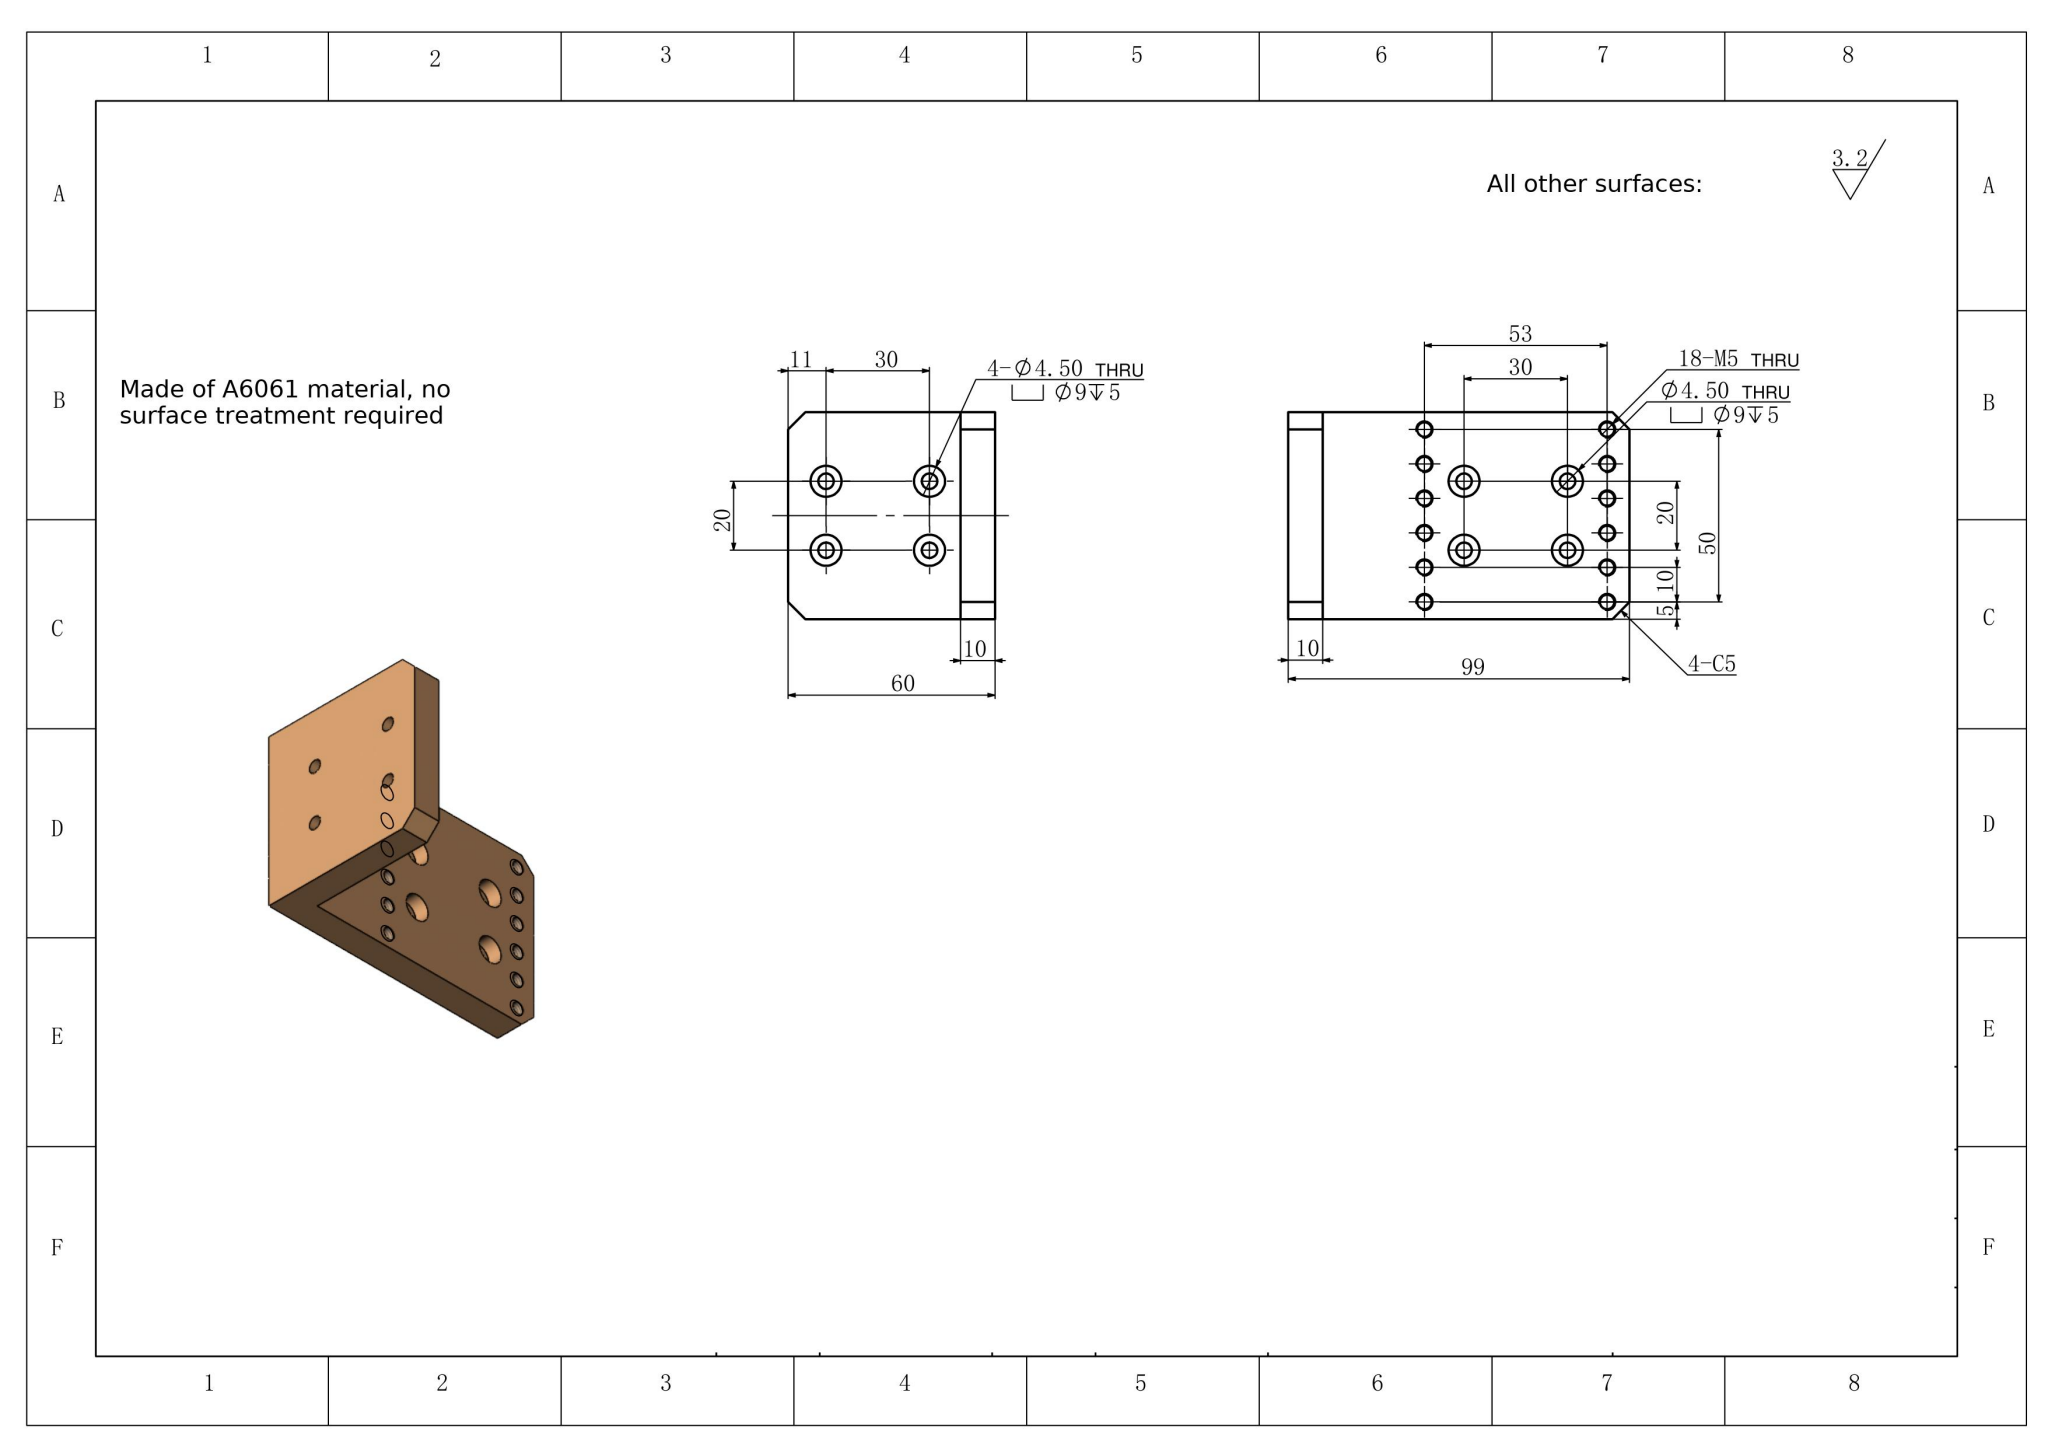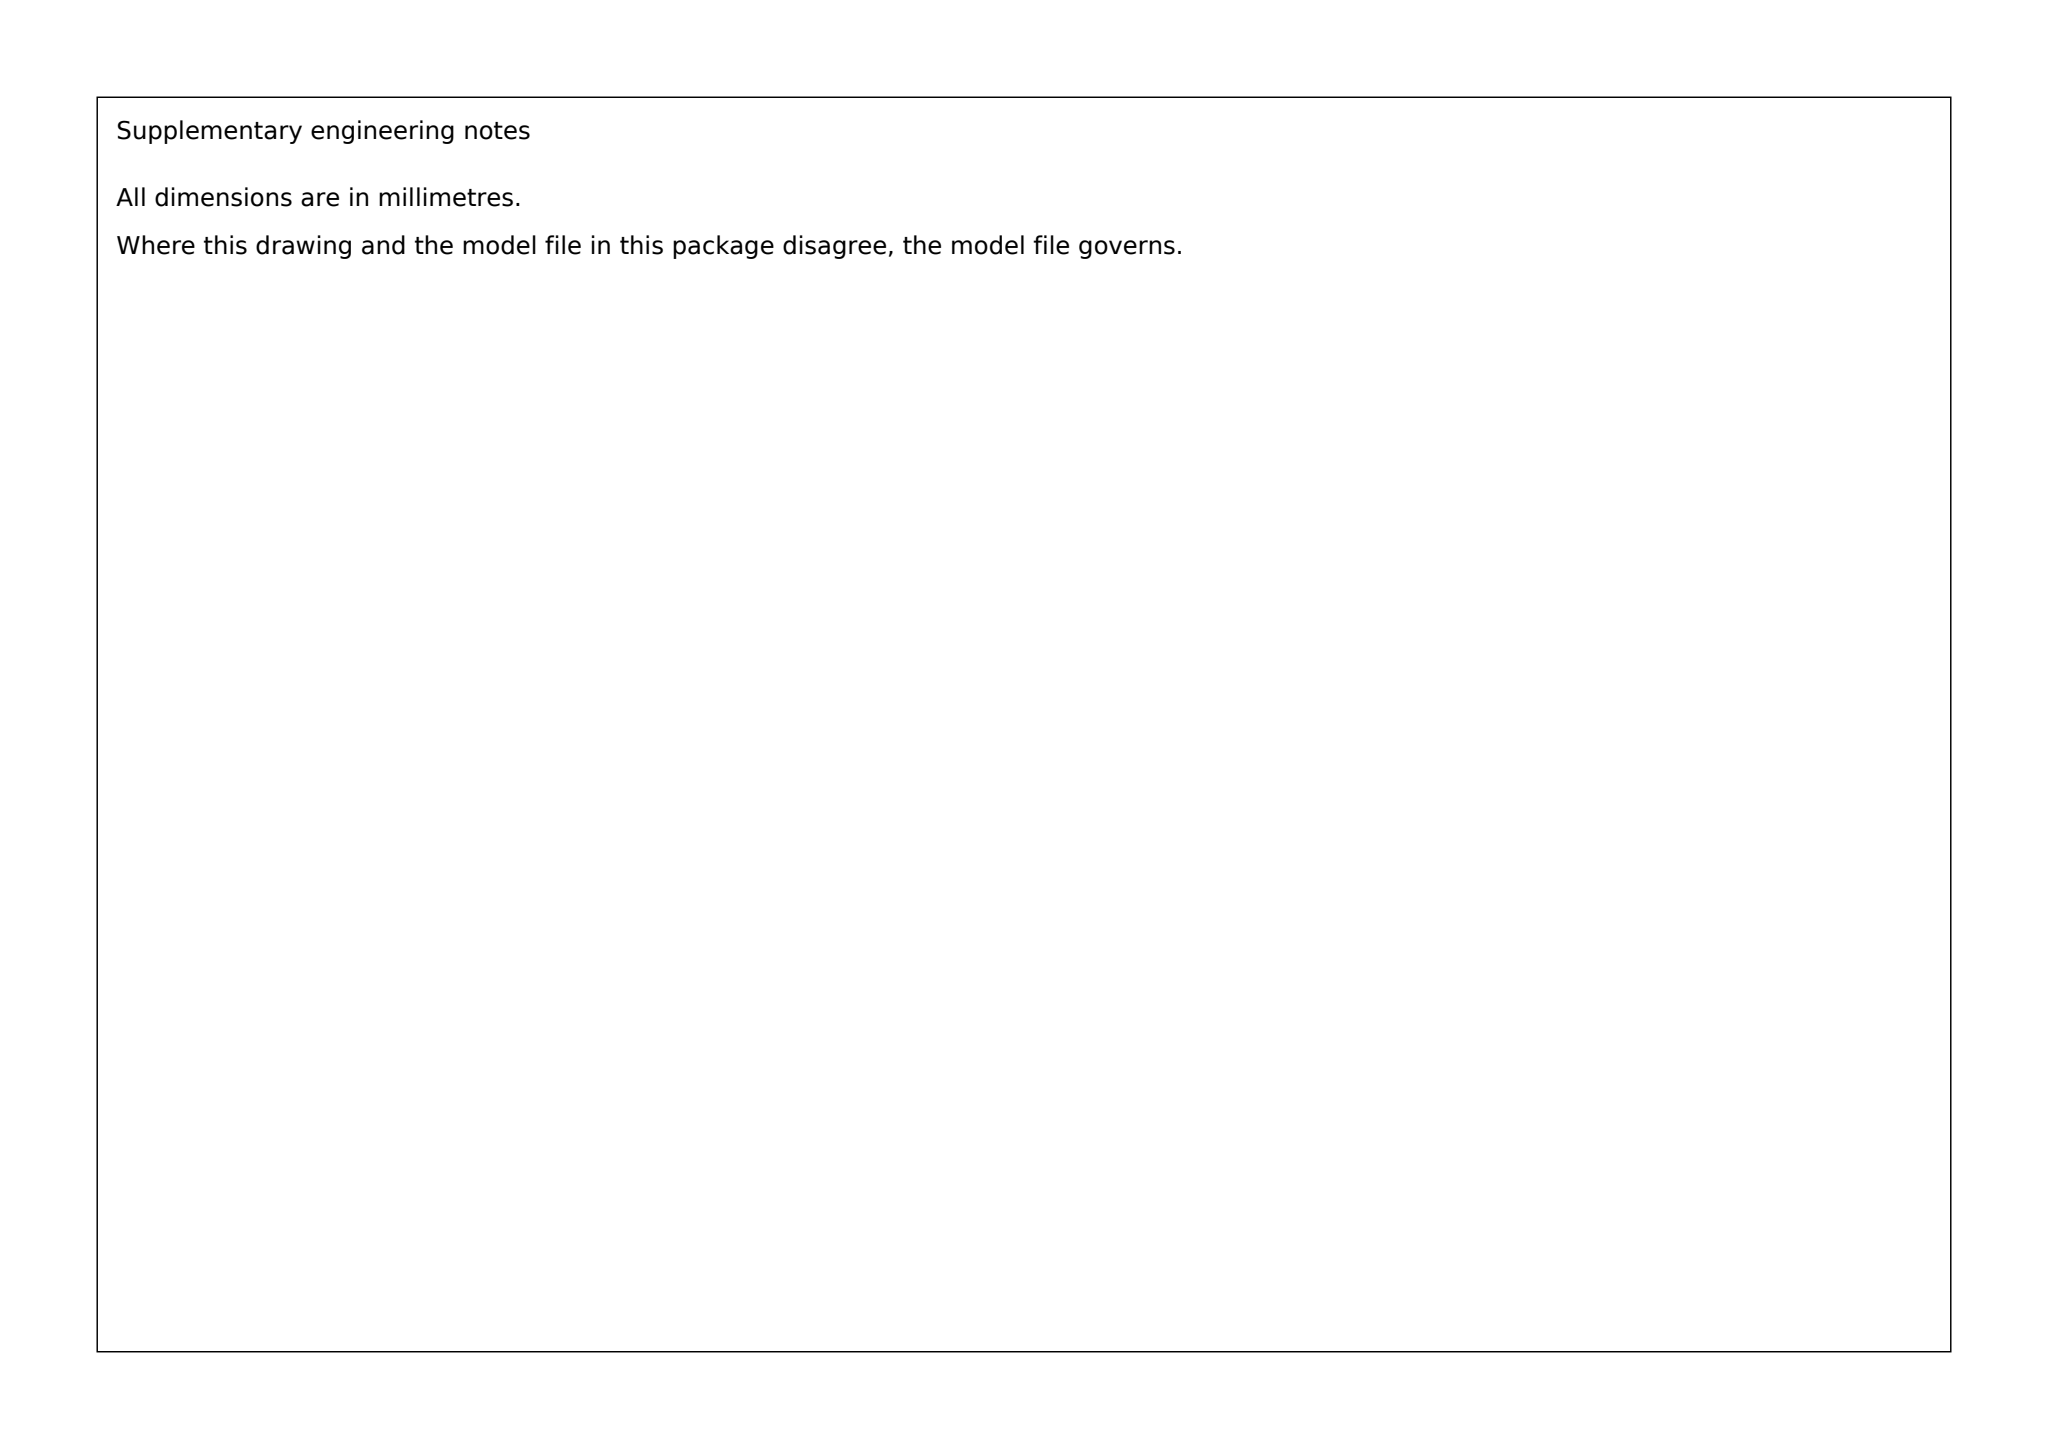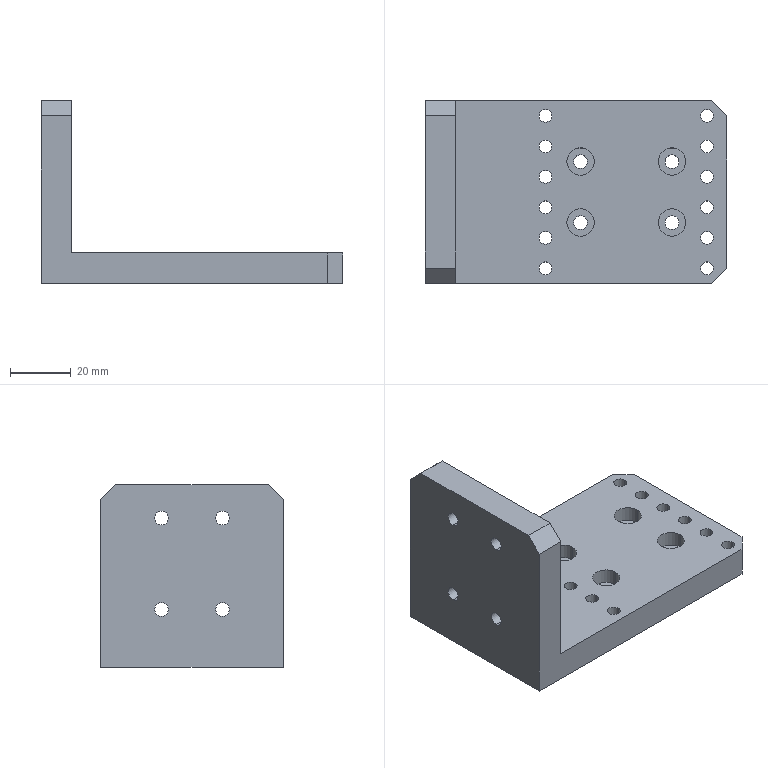Part | SolidWorks | mm | material A6061 | 1 solid | 76 faces | box 99 x 60 x 60 mm | volume 84057 mm3 | cylinder 56 | plane 20 | commonest cylinder face diameters 4.2 x24 4.5 x16 9 x16
build123d program:
from build123d import *

# Parameters (mm, degrees)
SKETCH1_W                  = 66
SKETCH1_H                  = 140
BOSS_EXTRUDE1_DEPTH        = 10
M5_TAPPED_HOLE1_AT_2_COUNT = 2
M5_TAPPED_HOLE1_AT_2_PITCH = 53
LPATTERN1_COUNT            = 14
LPATTERN1_PITCH            = 10
SKETCH4_R                  = 2.25
CUT_EXTRUDE1_DEPTH         = 79.032
SKETCH5_R                  = 4.5
CUT_EXTRUDE2_DEPTH         = 5
BOSS_EXTRUDE2_DEPTH        = 140
SKETCH7_R                  = 4.5
CUT_EXTRUDE3_DEPTH         = 5
SKETCH8_R                  = 2.25
CUT_EXTRUDE4_DEPTH         = 132.666
SKETCH9_W                  = 30
SKETCH9_H                  = 60
CUT_EXTRUDE5_DEPTH         = 129.144
FILLET1_R                  = 10
CUT_EXTRUDE6_DEPTH         = 109.425
SKETCH11_W                 = 117.715
SKETCH11_H                 = 97.512
CUT_EXTRUDE7_DEPTH         = 136.281
CHAMFER1_SIZE              = 5


with BuildPart() as part:
    # Sketch1 → Boss-Extrude1 (new body)
    with BuildSketch(Plane.XY):
        Rectangle(SKETCH1_W, SKETCH1_H)
    extrude(amount=BOSS_EXTRUDE1_DEPTH)

    # Sketch3 → M5 Tapped Hole1 (revolve, cut)
    with BuildSketch(Plane(origin=(-26.5, 65, 10), x_dir=(0, -1, 0), z_dir=(1, 0, 0))):
        Polygon((0, 0), (0, 17.662), (2.1, 16.4), (2.1, 0), align=None)
    m5_tapped_hole1 = revolve(axis=Axis((-26.5, 65, 16.35), (0, 0, -1)), mode=Mode.SUBTRACT)

    # M5 Tapped Hole1 at 2: M5 Tapped Hole1 ×2
    with Locations(*[(i * M5_TAPPED_HOLE1_AT_2_PITCH, 0, 0) for i in range(1, M5_TAPPED_HOLE1_AT_2_COUNT)]):
        add(m5_tapped_hole1, mode=Mode.SUBTRACT)

    # LPattern1: M5 Tapped Hole1 ×14
    with Locations(*[(0, -i * LPATTERN1_PITCH, 0) for i in range(1, LPATTERN1_COUNT)]):
        add(m5_tapped_hole1, mode=Mode.SUBTRACT)

    # LPattern1 copy 1 sketch → LPattern1 copy 1 (revolve, cut)
    with BuildSketch(Plane(origin=(26.5, 55, 10), x_dir=(0, -1, 0), z_dir=(1, 0, 0))):
        Polygon((0, 0), (0, 17.662), (2.1, 16.4), (2.1, 0), align=None)
    revolve(axis=Axis((26.5, 55, 16.35), (0, 0, -1)), mode=Mode.SUBTRACT)

    # LPattern1 copy 2 sketch → LPattern1 copy 2 (revolve, cut)
    with BuildSketch(Plane(origin=(26.5, 45, 10), x_dir=(0, -1, 0), z_dir=(1, 0, 0))):
        Polygon((0, 0), (0, 17.662), (2.1, 16.4), (2.1, 0), align=None)
    revolve(axis=Axis((26.5, 45, 16.35), (0, 0, -1)), mode=Mode.SUBTRACT)

    # LPattern1 copy 3 sketch → LPattern1 copy 3 (revolve, cut)
    with BuildSketch(Plane(origin=(26.5, 35, 10), x_dir=(0, -1, 0), z_dir=(1, 0, 0))):
        Polygon((0, 0), (0, 17.662), (2.1, 16.4), (2.1, 0), align=None)
    revolve(axis=Axis((26.5, 35, 16.35), (0, 0, -1)), mode=Mode.SUBTRACT)

    # LPattern1 copy 4 sketch → LPattern1 copy 4 (revolve, cut)
    with BuildSketch(Plane(origin=(26.5, 25, 10), x_dir=(0, -1, 0), z_dir=(1, 0, 0))):
        Polygon((0, 0), (0, 17.662), (2.1, 16.4), (2.1, 0), align=None)
    revolve(axis=Axis((26.5, 25, 16.35), (0, 0, -1)), mode=Mode.SUBTRACT)

    # LPattern1 copy 5 sketch → LPattern1 copy 5 (revolve, cut)
    with BuildSketch(Plane(origin=(26.5, 15, 10), x_dir=(0, -1, 0), z_dir=(1, 0, 0))):
        Polygon((0, 0), (0, 17.662), (2.1, 16.4), (2.1, 0), align=None)
    revolve(axis=Axis((26.5, 15, 16.35), (0, 0, -1)), mode=Mode.SUBTRACT)

    # LPattern1 copy 6 sketch → LPattern1 copy 6 (revolve, cut)
    with BuildSketch(Plane(origin=(26.5, 5, 10), x_dir=(0, -1, 0), z_dir=(1, 0, 0))):
        Polygon((0, 0), (0, 17.662), (2.1, 16.4), (2.1, 0), align=None)
    revolve(axis=Axis((26.5, 5, 16.35), (0, 0, -1)), mode=Mode.SUBTRACT)

    # LPattern1 copy 7 sketch → LPattern1 copy 7 (revolve, cut)
    with BuildSketch(Plane(origin=(26.5, -5, 10), x_dir=(0, -1, 0), z_dir=(1, 0, 0))):
        Polygon((0, 0), (0, 17.662), (2.1, 16.4), (2.1, 0), align=None)
    revolve(axis=Axis((26.5, -5, 16.35), (0, 0, -1)), mode=Mode.SUBTRACT)

    # LPattern1 copy 8 sketch → LPattern1 copy 8 (revolve, cut)
    with BuildSketch(Plane(origin=(26.5, -15, 10), x_dir=(0, -1, 0), z_dir=(1, 0, 0))):
        Polygon((0, 0), (0, 17.662), (2.1, 16.4), (2.1, 0), align=None)
    revolve(axis=Axis((26.5, -15, 16.35), (0, 0, -1)), mode=Mode.SUBTRACT)

    # LPattern1 copy 9 sketch → LPattern1 copy 9 (revolve, cut)
    with BuildSketch(Plane(origin=(26.5, -25, 10), x_dir=(0, -1, 0), z_dir=(1, 0, 0))):
        Polygon((0, 0), (0, 17.662), (2.1, 16.4), (2.1, 0), align=None)
    revolve(axis=Axis((26.5, -25, 16.35), (0, 0, -1)), mode=Mode.SUBTRACT)

    # LPattern1 copy 10 sketch → LPattern1 copy 10 (revolve, cut)
    with BuildSketch(Plane(origin=(26.5, -35, 10), x_dir=(0, -1, 0), z_dir=(1, 0, 0))):
        Polygon((0, 0), (0, 17.662), (2.1, 16.4), (2.1, 0), align=None)
    revolve(axis=Axis((26.5, -35, 16.35), (0, 0, -1)), mode=Mode.SUBTRACT)

    # LPattern1 copy 11 sketch → LPattern1 copy 11 (revolve, cut)
    with BuildSketch(Plane(origin=(26.5, -45, 10), x_dir=(0, -1, 0), z_dir=(1, 0, 0))):
        Polygon((0, 0), (0, 17.662), (2.1, 16.4), (2.1, 0), align=None)
    revolve(axis=Axis((26.5, -45, 16.35), (0, 0, -1)), mode=Mode.SUBTRACT)

    # LPattern1 copy 12 sketch → LPattern1 copy 12 (revolve, cut)
    with BuildSketch(Plane(origin=(26.5, -55, 10), x_dir=(0, -1, 0), z_dir=(1, 0, 0))):
        Polygon((0, 0), (0, 17.662), (2.1, 16.4), (2.1, 0), align=None)
    revolve(axis=Axis((26.5, -55, 16.35), (0, 0, -1)), mode=Mode.SUBTRACT)

    # LPattern1 copy 13 sketch → LPattern1 copy 13 (revolve, cut)
    with BuildSketch(Plane(origin=(26.5, -65, 10), x_dir=(0, -1, 0), z_dir=(1, 0, 0))):
        Polygon((0, 0), (0, 17.662), (2.1, 16.4), (2.1, 0), align=None)
    revolve(axis=Axis((26.5, -65, 16.35), (0, 0, -1)), mode=Mode.SUBTRACT)

    # Sketch4 → Cut-Extrude1 (cut, through all)
    with BuildSketch(Plane.XY.offset(10)):
        with Locations((-15, -30)):
            Circle(SKETCH4_R)
        with Locations((15, -30)):
            Circle(SKETCH4_R)
        with Locations((-15, -50)):
            Circle(SKETCH4_R)
        with Locations((15, -50)):
            Circle(SKETCH4_R)
    extrude(amount=-CUT_EXTRUDE1_DEPTH, mode=Mode.SUBTRACT)

    # Sketch5 → Cut-Extrude2 (cut)
    with BuildSketch(Plane.XY.offset(10)):
        with Locations((-15, -30)):
            Circle(SKETCH5_R)
        with Locations((-15, -50)):
            Circle(SKETCH5_R)
        with Locations((15, -30)):
            Circle(SKETCH5_R)
        with Locations((15, -50)):
            Circle(SKETCH5_R)
    extrude(amount=-CUT_EXTRUDE2_DEPTH, mode=Mode.SUBTRACT)

    # Sketch6 → Boss-Extrude2 (add)
    with BuildSketch(Plane(origin=(0, 70, 0), x_dir=(1, 0, 0), z_dir=(0, 1, 0))):
        Polygon((-33, 0), (-33, -10), (-56, -10), (-56, -60), (-66, -60), (-66, 0), align=None)
    extrude(amount=-BOSS_EXTRUDE2_DEPTH)

    # Sketch7 → Cut-Extrude3 (cut)
    with BuildSketch(Plane(origin=(-56, 0, 0), x_dir=(0, 0, -1), z_dir=(1, 0, 0))):
        with Locations((-49, -30)):
            Circle(SKETCH7_R)
        with Locations((-19, -30)):
            Circle(SKETCH7_R)
        with Locations((-19, -50)):
            Circle(SKETCH7_R)
        with Locations((-49, -50)):
            Circle(SKETCH7_R)
    extrude(amount=-CUT_EXTRUDE3_DEPTH, mode=Mode.SUBTRACT)

    # Sketch8 → Cut-Extrude4 (cut, through all)
    with BuildSketch(Plane(origin=(-61, 0, 0), x_dir=(0, 0, -1), z_dir=(1, 0, 0))):
        with Locations((-49, -30)):
            Circle(SKETCH8_R)
        with Locations((-19, -30)):
            Circle(SKETCH8_R)
        with Locations((-49, -50)):
            Circle(SKETCH8_R)
        with Locations((-19, -50)):
            Circle(SKETCH8_R)
    extrude(amount=-CUT_EXTRUDE4_DEPTH, mode=Mode.SUBTRACT)

    # Sketch9 → Cut-Extrude5 (cut, through all)
    with BuildSketch(Plane(origin=(-56, 0, 0), x_dir=(0, 0, -1), z_dir=(1, 0, 0))):
        with Locations((-35, 25)):
            Rectangle(SKETCH9_W, SKETCH9_H)
    extrude(amount=-CUT_EXTRUDE5_DEPTH, mode=Mode.SUBTRACT)

    # Fillet1
    fillet1_edges = [part.edges().sort_by_distance(p)[0] for p in [
        (-61, 55, 20),
        (-61, -5, 20),
        (-61, -5, 50),
        (-61, 55, 50),
    ]]
    fillet(fillet1_edges, radius=FILLET1_R)

    # Sketch10 → Cut-Extrude6 (cut, through all)
    with BuildSketch(Plane.XY.offset(10)):
        with BuildLine():
            Line((6.5, -5), (-6.5, -5))
            ThreePointArc((-6.5, -5), (-10.743, -3.243), (-12.5, 1))
            Line((-12.5, 1), (-12.5, 49))
            ThreePointArc((-12.5, 49), (-10.743, 53.243), (-6.5, 55))
            Line((-6.5, 55), (6.5, 55))
            ThreePointArc((6.5, 55), (10.743, 53.243), (12.5, 49))
            Line((12.5, 49), (12.5, 1))
            ThreePointArc((12.5, 1), (10.743, -3.243), (6.5, -5))
        make_face()
    extrude(amount=-CUT_EXTRUDE6_DEPTH, mode=Mode.SUBTRACT)

    # Sketch11 → Cut-Extrude7 (cut, through all)
    with BuildSketch(Plane.ZY.offset(66)):
        with Locations((33.176, 38.756)):
            Rectangle(SKETCH11_W, SKETCH11_H)
    extrude(amount=-CUT_EXTRUDE7_DEPTH, mode=Mode.SUBTRACT)

    # Chamfer1
    chamfer1_edges = [part.edges().sort_by_distance(p)[0] for p in [
        (-61, -70, 60),
        (33, -10, 5),
        (-61, -10, 60),
        (33, -70, 5),
    ]]
    chamfer(chamfer1_edges, length=CHAMFER1_SIZE)


solid = part.part